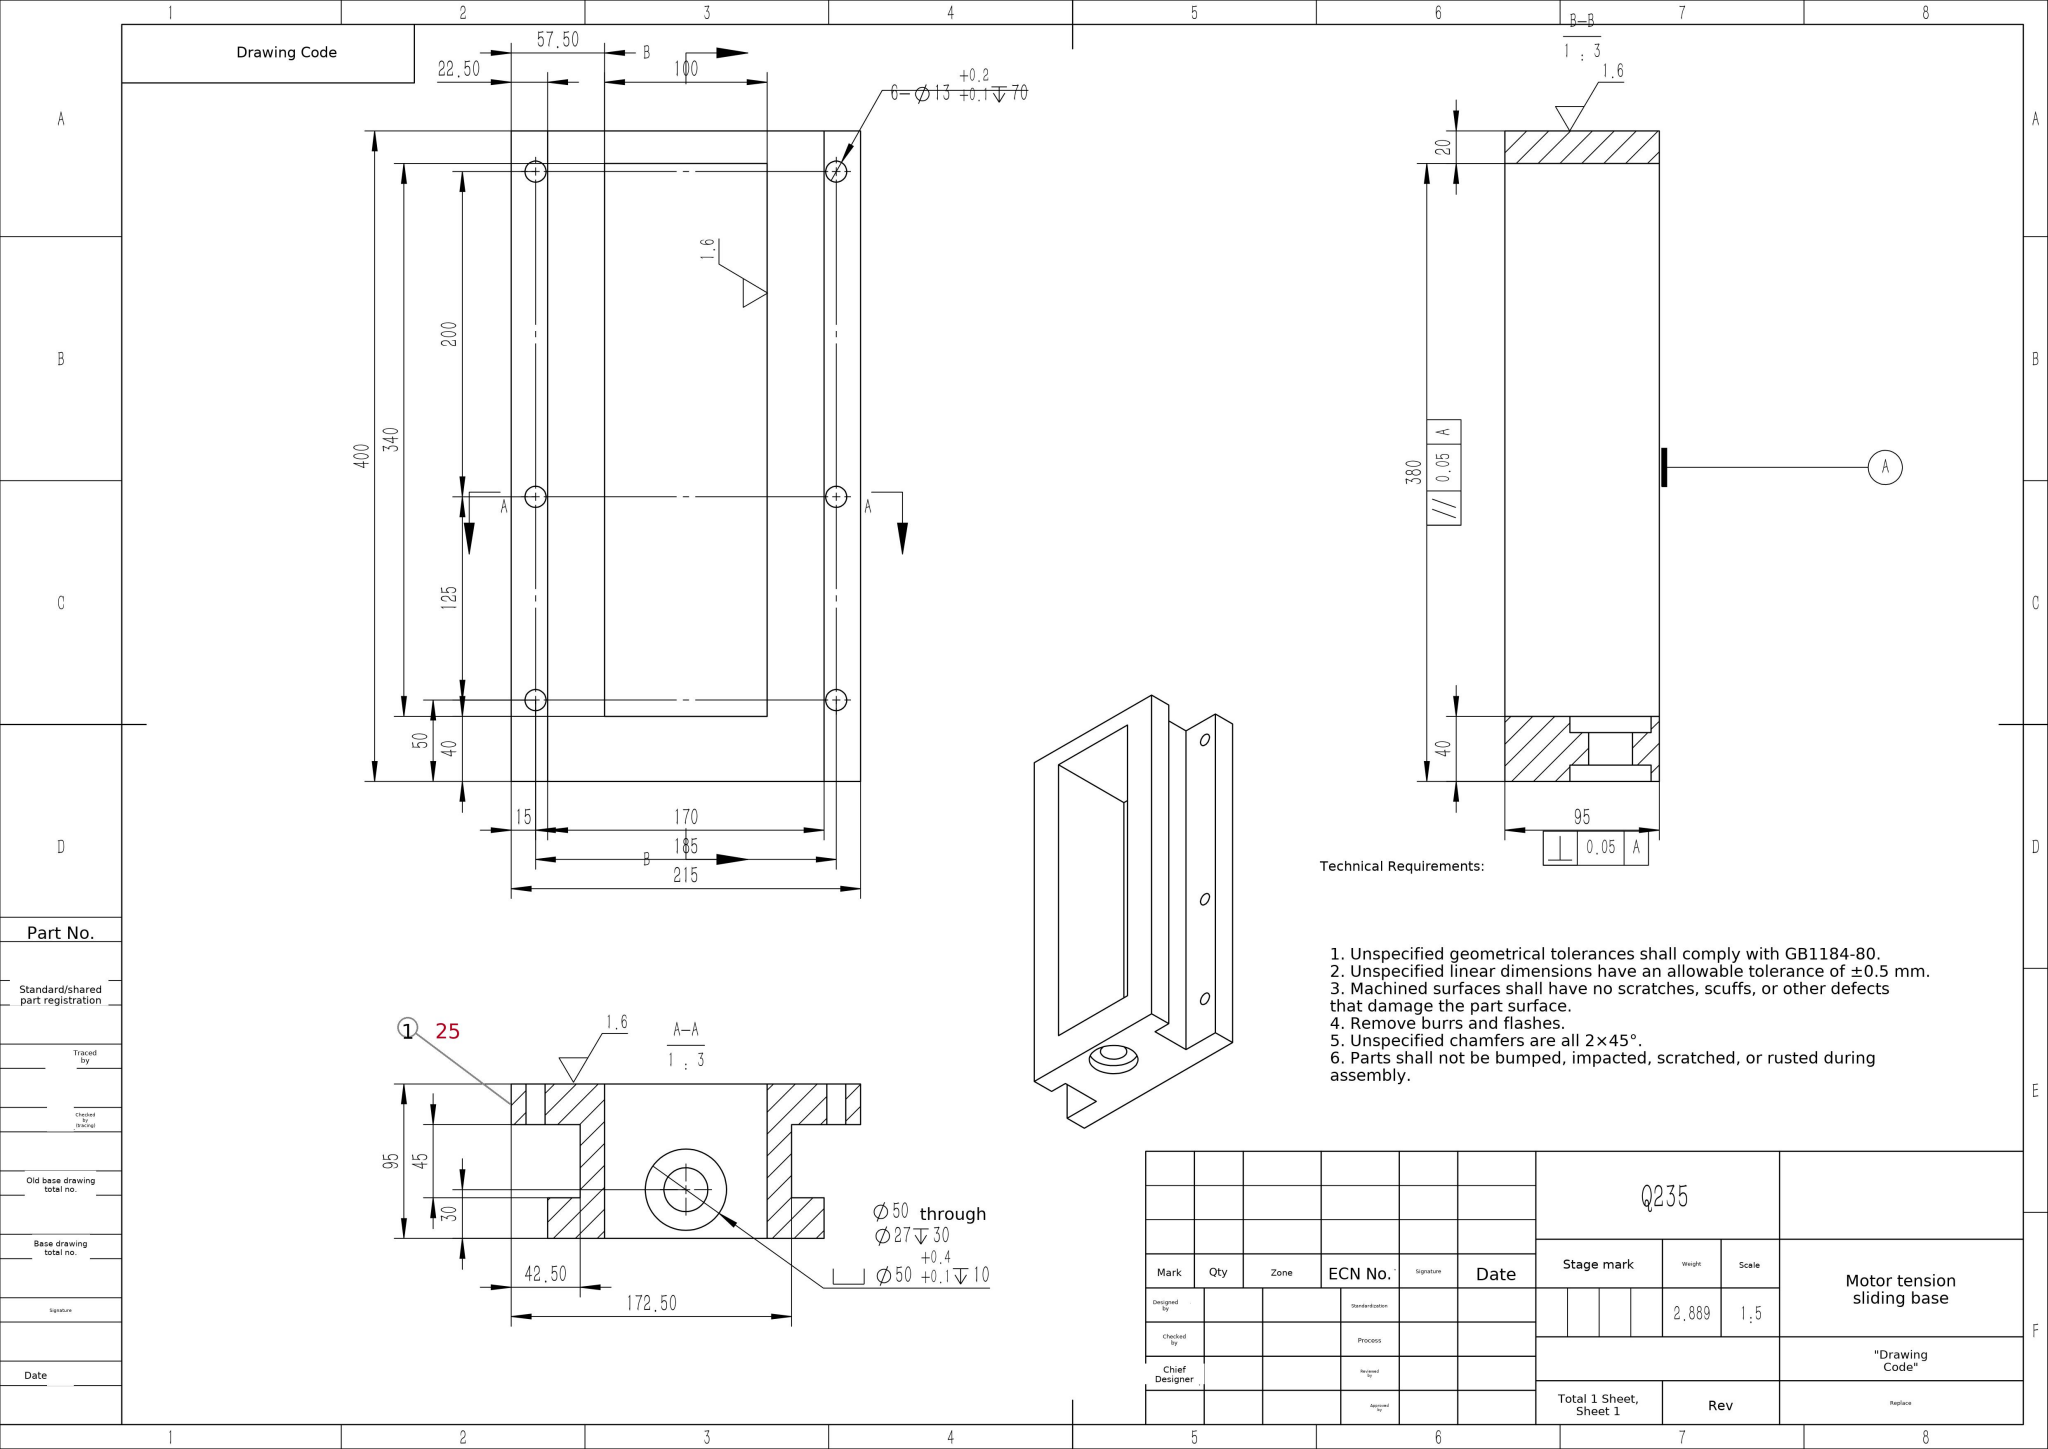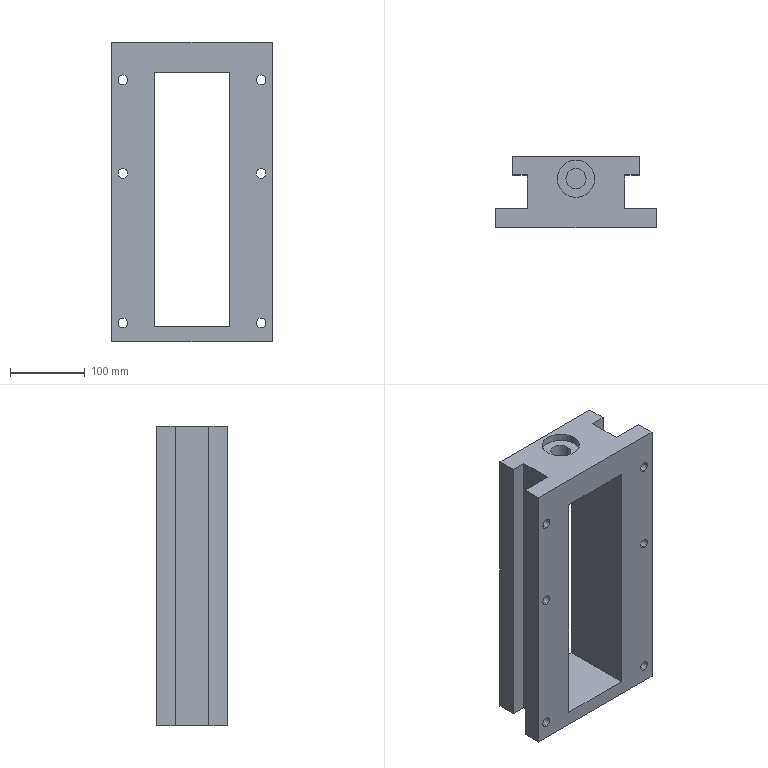Part | SolidWorks | mm | material Q235 | 1 solid | 38 faces | box 215 x 95 x 400 mm | volume 2889369 mm3 | plane 20 | cylinder 18 | commonest cylinder face diameters 13 x12 50 x4 27 x2
build123d program:
from build123d import *

# Parameters (mm, degrees)
BOSS_EXTRUDE1_DEPTH            = 400
CUT_EXTRUDE1_REACH             = 426.949
SKETCH2_W                      = 100
SKETCH2_H                      = 340
CUT_EXTRUDE2_REACH             = 426.949
SKETCH3_R                      = 13.5
SKETCH4_2_R                    = 25
CUT_EXTRUDE3_DEPTH             = 10
CUT_EXTRUDE4_START             = -30
SKETCH4_2_2_R                  = 25
CUT_EXTRUDE4_DEPTH             = 10
F_13_0_13_DIAMETER_HOLE1_D     = 13
F_13_0_13_DIAMETER_HOLE1_DEPTH = 70
F_13_0_13_DIAMETER_HOLE1_TIP   = 3.906


with BuildPart() as part:
    # Sketch1 → Boss-Extrude1 (new body)
    with BuildSketch(Plane.XY):
        Polygon((-107.5, 0), (107.5, 0), (107.5, 25), (65, 25), (65, 70), (85, 70), (85, 95), (-85, 95), (-85, 70), (-65, 70), (-65, 25), (-107.5, 25), align=None)
    extrude(amount=BOSS_EXTRUDE1_DEPTH)

    # Sketch2 → Cut-Extrude1 (cut, up to next)
    with BuildSketch(Plane(origin=(0, 95, 0), x_dir=(1, 0, 0), z_dir=(0, 1, 0)), mode=Mode.PRIVATE) as cut_extrude1_sk1:
        with Locations((0, -190)):
            Rectangle(SKETCH2_W, SKETCH2_H)
    cut_extrude1_tool1 = extrude(cut_extrude1_sk1.sketch, amount=-CUT_EXTRUDE1_REACH, mode=Mode.PRIVATE) & part.part
    add(cut_extrude1_tool1.solids().sort_by_distance((0, 95, 190))[0], mode=Mode.SUBTRACT)

    # Sketch3 → Cut-Extrude2 (cut, up to next)
    with BuildSketch(Plane.XY.offset(400), mode=Mode.PRIVATE) as cut_extrude2_sk1:
        with Locations((0, 65)):
            Circle(SKETCH3_R)
    cut_extrude2_tool1 = extrude(cut_extrude2_sk1.sketch, amount=-CUT_EXTRUDE2_REACH, mode=Mode.PRIVATE) & part.part
    add(cut_extrude2_tool1.solids().sort_by_distance((0, 65, 400))[0], mode=Mode.SUBTRACT)

    # Sketch4_2 → Cut-Extrude3 (cut)
    with BuildSketch(Plane.XY.offset(400)):
        with Locations((0, 65)):
            Circle(SKETCH4_2_R)
    extrude(amount=-CUT_EXTRUDE3_DEPTH, mode=Mode.SUBTRACT)

    # Sketch4_2 2 → Cut-Extrude4 (cut)
    with BuildSketch(Plane.XY.offset(400).offset(CUT_EXTRUDE4_START)):
        with Locations((0, 65)):
            Circle(SKETCH4_2_2_R)
    extrude(amount=-CUT_EXTRUDE4_DEPTH, mode=Mode.SUBTRACT)

    # 13.0 _13_ Diameter Hole1
    with Locations(Plane(origin=(0, 25, 0), x_dir=(1, 0, 0), z_dir=(0, 1, 0))):
        with Locations((-92.5, -350), (92.5, -350), (-92.5, -225), (92.5, -225), (-92.5, -25), (92.5, -25)):
            Hole(F_13_0_13_DIAMETER_HOLE1_D / 2, depth=F_13_0_13_DIAMETER_HOLE1_DEPTH)
            with Locations((0, 0, -(F_13_0_13_DIAMETER_HOLE1_DEPTH + F_13_0_13_DIAMETER_HOLE1_TIP / 2))):  # 118° drill point
                Cone(0, F_13_0_13_DIAMETER_HOLE1_D / 2, F_13_0_13_DIAMETER_HOLE1_TIP, mode=Mode.SUBTRACT)


solid = part.part